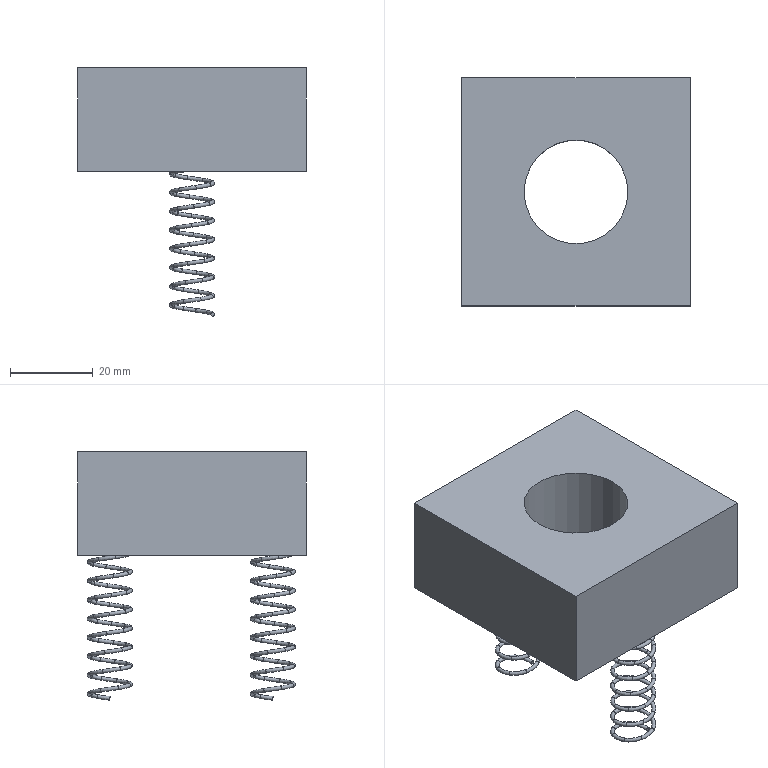Component | NX | PADS | 3 solids | 199 faces | volume 59012 mm3 | torus 184 | plane 10 | cylinder 3 | cone 2 | commonest cylinder face diameters 12 x2 25.025 x1